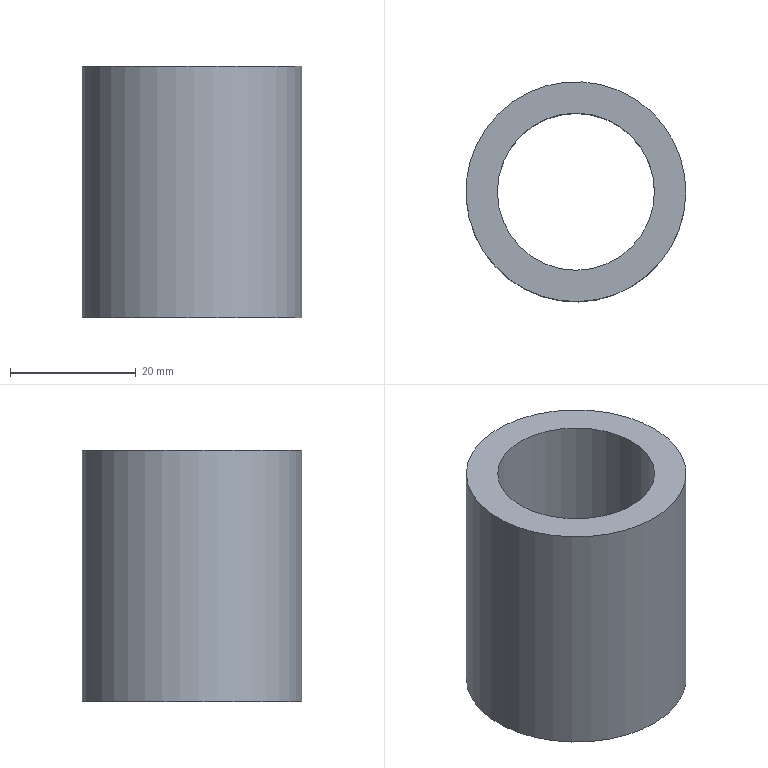Component | NX | SLIDER_FRAME_CONN_RING_2 | 1 solid | 4 faces | box 35 x 35 x 40 mm | volume 18850 mm3 | cylinder 2 | plane 2 | commonest cylinder face diameters 35 x1 25 x1
STEP:
#1=CARTESIAN_POINT('',(0.,0.,0.));
#2=DIRECTION('',(0.,0.,1.));
#3=DIRECTION('',(1.,0.,0.));
#4=AXIS2_PLACEMENT_3D('',#1,#2,#3);
#5=CARTESIAN_POINT('',(-276.192,1067.527,215.));
#6=VERTEX_POINT('',#5);
#7=CARTESIAN_POINT('',(-263.818,1055.152,215.));
#8=DIRECTION('',(0.,0.,-1.));
#9=DIRECTION('',(-0.7071,0.7071,0.));
#10=AXIS2_PLACEMENT_3D('',#7,#8,#9);
#11=CIRCLE('',#10,17.5);
#12=CARTESIAN_POINT('',(-263.818,1055.152,215.));
#13=DIRECTION('',(0.,0.,-1.));
#14=DIRECTION('',(0.7071,-0.7071,0.));
#15=AXIS2_PLACEMENT_3D('',#12,#13,#14);
#16=CYLINDRICAL_SURFACE('',#15,17.5);
#17=CARTESIAN_POINT('',(3.142,0.));
#18=DIRECTION('',(1.,0.));
#19=VECTOR('',#18,1.);
#20=LINE('',#17,#19);
#21=(GEOMETRIC_REPRESENTATION_CONTEXT(2)PARAMETRIC_REPRESENTATION_CONTEXT()REPRESENTATION_CONTEXT('',''));
#22=DEFINITIONAL_REPRESENTATION('',(#20),#21);
#23=PCURVE('',#16,#22);
#24=CARTESIAN_POINT('',(-263.818,1055.152,215.));
#25=DIRECTION('',(0.,0.,-1.));
#26=DIRECTION('',(0.7071,-0.7071,0.));
#27=AXIS2_PLACEMENT_3D('',#24,#25,#26);
#28=PLANE('',#27);
#29=CARTESIAN_POINT('',(0.,0.));
#30=DIRECTION('',(-1.,0.));
#31=AXIS2_PLACEMENT_2D('',#29,#30);
#32=CIRCLE('',#31,17.5);
#33=(GEOMETRIC_REPRESENTATION_CONTEXT(2)PARAMETRIC_REPRESENTATION_CONTEXT()REPRESENTATION_CONTEXT('',''));
#34=DEFINITIONAL_REPRESENTATION('',(#32),#33);
#35=PCURVE('',#28,#34);
#36=SURFACE_CURVE('',#11,(#23,#35),.PCURVE_S1.);
#37=EDGE_CURVE('',#6,#6,#36,.T.);
#38=ORIENTED_EDGE('',*,*,#37,.T.);
#39=CARTESIAN_POINT('',(-276.192,1067.527,175.));
#40=VERTEX_POINT('',#39);
#41=CARTESIAN_POINT('',(-276.192,1067.527,215.));
#42=CARTESIAN_POINT('',(-276.192,1067.527,175.));
#43=B_SPLINE_CURVE_WITH_KNOTS('',1,(#41,#42),.UNSPECIFIED.,.F.,.F.,(2,2),(0.,40.),.PIECEWISE_BEZIER_KNOTS.);
#44=CARTESIAN_POINT('',(9.425,0.));
#45=DIRECTION('',(0.,1.));
#46=VECTOR('',#45,1.);
#47=LINE('',#44,#46);
#48=(GEOMETRIC_REPRESENTATION_CONTEXT(2)PARAMETRIC_REPRESENTATION_CONTEXT()REPRESENTATION_CONTEXT('',''));
#49=DEFINITIONAL_REPRESENTATION('',(#47),#48);
#50=PCURVE('',#16,#49);
#51=CARTESIAN_POINT('',(3.142,0.));
#52=DIRECTION('',(0.,1.));
#53=VECTOR('',#52,1.);
#54=LINE('',#51,#53);
#55=(GEOMETRIC_REPRESENTATION_CONTEXT(2)PARAMETRIC_REPRESENTATION_CONTEXT()REPRESENTATION_CONTEXT('',''));
#56=DEFINITIONAL_REPRESENTATION('',(#54),#55);
#57=PCURVE('',#16,#56);
#58=SEAM_CURVE('',#43,(#50,#57),.PCURVE_S1.);
#59=EDGE_CURVE('',#6,#40,#58,.T.);
#60=ORIENTED_EDGE('',*,*,#59,.T.);
#61=CARTESIAN_POINT('',(-263.818,1055.152,175.));
#62=DIRECTION('',(0.,0.,-1.));
#63=DIRECTION('',(-0.7071,0.7071,0.));
#64=AXIS2_PLACEMENT_3D('',#61,#62,#63);
#65=CIRCLE('',#64,17.5);
#66=CARTESIAN_POINT('',(3.142,40.));
#67=DIRECTION('',(1.,0.));
#68=VECTOR('',#67,1.);
#69=LINE('',#66,#68);
#70=(GEOMETRIC_REPRESENTATION_CONTEXT(2)PARAMETRIC_REPRESENTATION_CONTEXT()REPRESENTATION_CONTEXT('',''));
#71=DEFINITIONAL_REPRESENTATION('',(#69),#70);
#72=PCURVE('',#16,#71);
#73=CARTESIAN_POINT('',(-263.818,1055.152,175.));
#74=DIRECTION('',(0.,0.,-1.));
#75=DIRECTION('',(0.7071,-0.7071,0.));
#76=AXIS2_PLACEMENT_3D('',#73,#74,#75);
#77=PLANE('',#76);
#78=CARTESIAN_POINT('',(0.,0.));
#79=DIRECTION('',(-1.,0.));
#80=AXIS2_PLACEMENT_2D('',#78,#79);
#81=CIRCLE('',#80,17.5);
#82=(GEOMETRIC_REPRESENTATION_CONTEXT(2)PARAMETRIC_REPRESENTATION_CONTEXT()REPRESENTATION_CONTEXT('',''));
#83=DEFINITIONAL_REPRESENTATION('',(#81),#82);
#84=PCURVE('',#77,#83);
#85=SURFACE_CURVE('',#65,(#72,#84),.PCURVE_S1.);
#86=EDGE_CURVE('',#40,#40,#85,.T.);
#87=ORIENTED_EDGE('',*,*,#86,.F.);
#88=ORIENTED_EDGE('',*,*,#59,.F.);
#89=EDGE_LOOP('',(#38,#60,#87,#88));
#90=FACE_BOUND('',#89,.T.);
#91=ADVANCED_FACE('',(#90),#16,.T.);
#92=CARTESIAN_POINT('',(-272.657,1063.991,215.));
#93=VERTEX_POINT('',#92);
#94=CARTESIAN_POINT('',(-263.818,1055.152,215.));
#95=DIRECTION('',(0.,0.,-1.));
#96=DIRECTION('',(-0.7071,0.7071,0.));
#97=AXIS2_PLACEMENT_3D('',#94,#95,#96);
#98=CIRCLE('',#97,12.5);
#99=CARTESIAN_POINT('',(-263.818,1055.152,215.));
#100=DIRECTION('',(0.,0.,-1.));
#101=DIRECTION('',(0.7071,-0.7071,0.));
#102=AXIS2_PLACEMENT_3D('',#99,#100,#101);
#103=CYLINDRICAL_SURFACE('',#102,12.5);
#104=CARTESIAN_POINT('',(3.142,0.));
#105=DIRECTION('',(1.,0.));
#106=VECTOR('',#105,1.);
#107=LINE('',#104,#106);
#108=(GEOMETRIC_REPRESENTATION_CONTEXT(2)PARAMETRIC_REPRESENTATION_CONTEXT()REPRESENTATION_CONTEXT('',''));
#109=DEFINITIONAL_REPRESENTATION('',(#107),#108);
#110=PCURVE('',#103,#109);
#111=CARTESIAN_POINT('',(0.,0.));
#112=DIRECTION('',(-1.,0.));
#113=AXIS2_PLACEMENT_2D('',#111,#112);
#114=CIRCLE('',#113,12.5);
#115=(GEOMETRIC_REPRESENTATION_CONTEXT(2)PARAMETRIC_REPRESENTATION_CONTEXT()REPRESENTATION_CONTEXT('',''));
#116=DEFINITIONAL_REPRESENTATION('',(#114),#115);
#117=PCURVE('',#28,#116);
#118=SURFACE_CURVE('',#98,(#110,#117),.PCURVE_S1.);
#119=EDGE_CURVE('',#93,#93,#118,.T.);
#120=ORIENTED_EDGE('',*,*,#119,.T.);
#121=CARTESIAN_POINT('',(-272.657,1063.991,175.));
#122=VERTEX_POINT('',#121);
#123=CARTESIAN_POINT('',(-272.657,1063.991,215.));
#124=CARTESIAN_POINT('',(-272.657,1063.991,175.));
#125=B_SPLINE_CURVE_WITH_KNOTS('',1,(#123,#124),.UNSPECIFIED.,.F.,.F.,(2,2),(0.,40.),.PIECEWISE_BEZIER_KNOTS.);
#126=CARTESIAN_POINT('',(9.425,0.));
#127=DIRECTION('',(0.,1.));
#128=VECTOR('',#127,1.);
#129=LINE('',#126,#128);
#130=(GEOMETRIC_REPRESENTATION_CONTEXT(2)PARAMETRIC_REPRESENTATION_CONTEXT()REPRESENTATION_CONTEXT('',''));
#131=DEFINITIONAL_REPRESENTATION('',(#129),#130);
#132=PCURVE('',#103,#131);
#133=CARTESIAN_POINT('',(3.142,0.));
#134=DIRECTION('',(0.,1.));
#135=VECTOR('',#134,1.);
#136=LINE('',#133,#135);
#137=(GEOMETRIC_REPRESENTATION_CONTEXT(2)PARAMETRIC_REPRESENTATION_CONTEXT()REPRESENTATION_CONTEXT('',''));
#138=DEFINITIONAL_REPRESENTATION('',(#136),#137);
#139=PCURVE('',#103,#138);
#140=SEAM_CURVE('',#125,(#132,#139),.PCURVE_S1.);
#141=EDGE_CURVE('',#93,#122,#140,.T.);
#142=ORIENTED_EDGE('',*,*,#141,.T.);
#143=CARTESIAN_POINT('',(-263.818,1055.152,175.));
#144=DIRECTION('',(0.,0.,-1.));
#145=DIRECTION('',(-0.7071,0.7071,0.));
#146=AXIS2_PLACEMENT_3D('',#143,#144,#145);
#147=CIRCLE('',#146,12.5);
#148=CARTESIAN_POINT('',(3.142,40.));
#149=DIRECTION('',(1.,0.));
#150=VECTOR('',#149,1.);
#151=LINE('',#148,#150);
#152=(GEOMETRIC_REPRESENTATION_CONTEXT(2)PARAMETRIC_REPRESENTATION_CONTEXT()REPRESENTATION_CONTEXT('',''));
#153=DEFINITIONAL_REPRESENTATION('',(#151),#152);
#154=PCURVE('',#103,#153);
#155=CARTESIAN_POINT('',(0.,0.));
#156=DIRECTION('',(-1.,0.));
#157=AXIS2_PLACEMENT_2D('',#155,#156);
#158=CIRCLE('',#157,12.5);
#159=(GEOMETRIC_REPRESENTATION_CONTEXT(2)PARAMETRIC_REPRESENTATION_CONTEXT()REPRESENTATION_CONTEXT('',''));
#160=DEFINITIONAL_REPRESENTATION('',(#158),#159);
#161=PCURVE('',#77,#160);
#162=SURFACE_CURVE('',#147,(#154,#161),.PCURVE_S1.);
#163=EDGE_CURVE('',#122,#122,#162,.T.);
#164=ORIENTED_EDGE('',*,*,#163,.F.);
#165=ORIENTED_EDGE('',*,*,#141,.F.);
#166=EDGE_LOOP('',(#120,#142,#164,#165));
#167=FACE_BOUND('',#166,.F.);
#168=ADVANCED_FACE('',(#167),#103,.F.);
#169=ORIENTED_EDGE('',*,*,#37,.F.);
#170=EDGE_LOOP('',(#169));
#171=FACE_BOUND('',#170,.T.);
#172=ORIENTED_EDGE('',*,*,#119,.T.);
#173=EDGE_LOOP('',(#172));
#174=FACE_BOUND('',#173,.T.);
#175=ADVANCED_FACE('',(#171,#174),#28,.F.);
#176=ORIENTED_EDGE('',*,*,#86,.T.);
#177=EDGE_LOOP('',(#176));
#178=FACE_BOUND('',#177,.T.);
#179=ORIENTED_EDGE('',*,*,#163,.F.);
#180=EDGE_LOOP('',(#179));
#181=FACE_BOUND('',#180,.T.);
#182=ADVANCED_FACE('',(#178,#181),#77,.T.);
#183=CLOSED_SHELL('',(#91,#168,#175,#182));
#184=MANIFOLD_SOLID_BREP('',#183);
#185=(LENGTH_UNIT()NAMED_UNIT(*)SI_UNIT(.MILLI.,.METRE.));
#186=UNCERTAINTY_MEASURE_WITH_UNIT(LENGTH_MEASURE(0.00001),#185,'','');
#187=(NAMED_UNIT(*)PLANE_ANGLE_UNIT()SI_UNIT($,.RADIAN.));
#188=(NAMED_UNIT(*)SI_UNIT($,.STERADIAN.)SOLID_ANGLE_UNIT());
#189=(GEOMETRIC_REPRESENTATION_CONTEXT(3)GLOBAL_UNCERTAINTY_ASSIGNED_CONTEXT((#186))GLOBAL_UNIT_ASSIGNED_CONTEXT((#185,#187,#188))REPRESENTATION_CONTEXT('',''));
#190=ADVANCED_BREP_SHAPE_REPRESENTATION('',(#4,#184),#189);